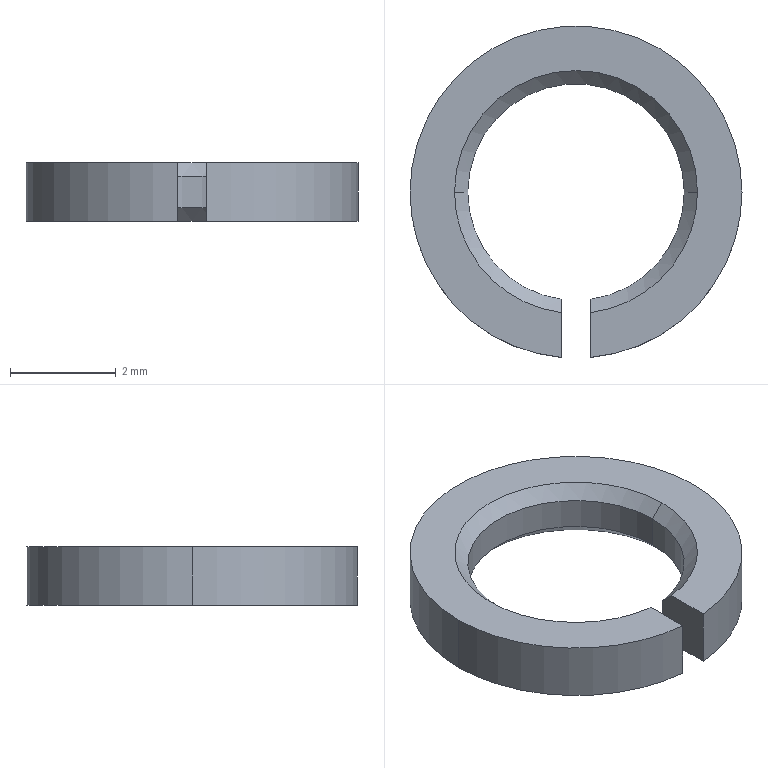Component | SolidWorks | GB_T93-1987StandardTypeSpringWasher4_1.1-6 | 1 solid | 16 faces | box 6.29 x 6.27 x 1.1 mm | volume 18 mm3 | cone 6 | cylinder 6 | plane 4 | commonest cylinder face diameters 4.1 x3 6.287 x3 | material 65Mn
build123d program:
from build123d import *

# Parameters (mm, degrees)
EXTRUDE1_DEPTH = 1.1
CHAMFER1_SIZE  = 0.25


with BuildPart() as part:
    # Sketch1 → Extrude1 (new body)
    with BuildSketch(Plane.XY):
        with BuildLine():
            Line((-0.275, 3.131), (-0.275, 2.031))
            ThreePointArc((-0.275, 2.031), (0, -2.05), (0.275, 2.031))
            Line((0.275, 2.031), (0.275, 3.131))
            ThreePointArc((0.275, 3.131), (0, -3.144), (-0.275, 3.131))
        make_face()
    extrude(amount=EXTRUDE1_DEPTH)

    # Chamfer1
    chamfer1_edges = [part.edges().sort_by_distance(p)[0] for p in [
        (0, -2.05, 1.1),
        (0, -2.05, 0),
    ]]
    chamfer(chamfer1_edges, length=CHAMFER1_SIZE)


solid = part.part

# Placed as in the assembly
solid = solid.moved(Location((58.994, 24.5, 13.9), (180, 0, 0)))
STEP:
#1=COLOUR_RGB('',0.7922,0.8196,0.9333);
#2=FILL_AREA_STYLE_COLOUR('',#1);
#3=FILL_AREA_STYLE('',(#2));
#4=SURFACE_STYLE_FILL_AREA(#3);
#5=SURFACE_SIDE_STYLE('',(#4));
#6=SURFACE_STYLE_USAGE(.BOTH.,#5);
#7=PRESENTATION_STYLE_ASSIGNMENT((#6));
#8=CARTESIAN_POINT('',(2.403,0.9646,0.5374));
#9=VERTEX_POINT('',#8);
#10=CARTESIAN_POINT('',(2.242,0.9646,0.5374));
#11=VERTEX_POINT('',#10);
#12=CARTESIAN_POINT('',(2.323,0.9646,0.5374));
#13=DIRECTION('',(0.,0.,1.));
#14=DIRECTION('',(1.,0.,0.));
#15=AXIS2_PLACEMENT_3D('',#12,#13,#14);
#16=CIRCLE('',#15,0.08071);
#17=EDGE_CURVE('',#9,#11,#16,.T.);
#18=ORIENTED_EDGE('',*,*,#17,.F.);
#19=CARTESIAN_POINT('',(2.413,0.9646,0.5472));
#20=VERTEX_POINT('',#19);
#21=CARTESIAN_POINT('',(2.403,0.9646,0.5374));
#22=DIRECTION('',(0.7071,0.,0.7071));
#23=VECTOR('',#22,39.37);
#24=LINE('',#21,#23);
#25=EDGE_CURVE('',#9,#20,#24,.T.);
#26=ORIENTED_EDGE('',*,*,#25,.T.);
#27=CARTESIAN_POINT('',(2.232,0.9646,0.5472));
#28=VERTEX_POINT('',#27);
#29=CARTESIAN_POINT('',(2.323,0.9646,0.5472));
#30=DIRECTION('',(0.,-0.,-1.));
#31=DIRECTION('',(1.,0.,0.));
#32=AXIS2_PLACEMENT_3D('',#29,#30,#31);
#33=CIRCLE('',#32,0.09055);
#34=EDGE_CURVE('',#28,#20,#33,.T.);
#35=ORIENTED_EDGE('',*,*,#34,.F.);
#36=CARTESIAN_POINT('',(2.242,0.9646,0.5374));
#37=DIRECTION('',(-0.7071,0.,0.7071));
#38=VECTOR('',#37,39.37);
#39=LINE('',#36,#38);
#40=EDGE_CURVE('',#11,#28,#39,.T.);
#41=ORIENTED_EDGE('',*,*,#40,.F.);
#42=EDGE_LOOP('',(#18,#26,#35,#41));
#43=FACE_OUTER_BOUND('',#42,.T.);
#44=CARTESIAN_POINT('',(2.323,0.9646,0.5374));
#45=DIRECTION('',(0.,0.,1.));
#46=DIRECTION('',(-1.,0.,0.));
#47=AXIS2_PLACEMENT_3D('',#44,#45,#46);
#48=CONICAL_SURFACE('',#47,0.08071,0.7854);
#49=ADVANCED_FACE('',(#43),#48,.F.);
#50=CARTESIAN_POINT('',(2.312,0.8846,0.5374));
#51=VERTEX_POINT('',#50);
#52=CARTESIAN_POINT('',(2.323,0.9646,0.5374));
#53=DIRECTION('',(0.,0.,1.));
#54=DIRECTION('',(1.,0.,0.));
#55=AXIS2_PLACEMENT_3D('',#52,#53,#54);
#56=CIRCLE('',#55,0.08071);
#57=EDGE_CURVE('',#11,#51,#56,.T.);
#58=ORIENTED_EDGE('',*,*,#57,.F.);
#59=ORIENTED_EDGE('',*,*,#40,.T.);
#60=CARTESIAN_POINT('',(2.312,0.8747,0.5472));
#61=VERTEX_POINT('',#60);
#62=CARTESIAN_POINT('',(2.323,0.9646,0.5472));
#63=DIRECTION('',(0.,-0.,-1.));
#64=DIRECTION('',(1.,0.,0.));
#65=AXIS2_PLACEMENT_3D('',#62,#63,#64);
#66=CIRCLE('',#65,0.09055);
#67=EDGE_CURVE('',#61,#28,#66,.T.);
#68=ORIENTED_EDGE('',*,*,#67,.F.);
#69=CARTESIAN_POINT('',(2.312,0.8846,0.5374));
#70=CARTESIAN_POINT('',(2.312,0.8813,0.5407));
#71=CARTESIAN_POINT('',(2.312,0.878,0.544));
#72=CARTESIAN_POINT('',(2.312,0.8747,0.5472));
#73=B_SPLINE_CURVE_WITH_KNOTS('',3,(#69,#70,#71,#72),.UNSPECIFIED.,.F.,.F.,(4,4),(0.,0.000355),.UNSPECIFIED.);
#74=EDGE_CURVE('',#51,#61,#73,.T.);
#75=ORIENTED_EDGE('',*,*,#74,.F.);
#76=EDGE_LOOP('',(#58,#59,#68,#75));
#77=FACE_OUTER_BOUND('',#76,.T.);
#78=CARTESIAN_POINT('',(2.323,0.9646,0.5374));
#79=DIRECTION('',(0.,0.,1.));
#80=DIRECTION('',(-1.,0.,0.));
#81=AXIS2_PLACEMENT_3D('',#78,#79,#80);
#82=CONICAL_SURFACE('',#81,0.08071,0.7854);
#83=ADVANCED_FACE('',(#77),#82,.F.);
#84=CARTESIAN_POINT('',(2.242,0.9646,0.5138));
#85=VERTEX_POINT('',#84);
#86=CARTESIAN_POINT('',(2.403,0.9646,0.5138));
#87=VERTEX_POINT('',#86);
#88=CARTESIAN_POINT('',(2.323,0.9646,0.5138));
#89=DIRECTION('',(0.,-0.,-1.));
#90=DIRECTION('',(1.,0.,0.));
#91=AXIS2_PLACEMENT_3D('',#88,#89,#90);
#92=CIRCLE('',#91,0.08071);
#93=EDGE_CURVE('',#85,#87,#92,.T.);
#94=ORIENTED_EDGE('',*,*,#93,.F.);
#95=CARTESIAN_POINT('',(2.232,0.9646,0.5039));
#96=VERTEX_POINT('',#95);
#97=CARTESIAN_POINT('',(2.232,0.9646,0.5039));
#98=DIRECTION('',(-0.7071,-0.,-0.7071));
#99=VECTOR('',#98,39.37);
#100=LINE('',#97,#99);
#101=EDGE_CURVE('',#85,#96,#100,.T.);
#102=ORIENTED_EDGE('',*,*,#101,.T.);
#103=CARTESIAN_POINT('',(2.413,0.9646,0.5039));
#104=VERTEX_POINT('',#103);
#105=CARTESIAN_POINT('',(2.323,0.9646,0.5039));
#106=DIRECTION('',(0.,0.,1.));
#107=DIRECTION('',(1.,0.,0.));
#108=AXIS2_PLACEMENT_3D('',#105,#106,#107);
#109=CIRCLE('',#108,0.09055);
#110=EDGE_CURVE('',#104,#96,#109,.T.);
#111=ORIENTED_EDGE('',*,*,#110,.F.);
#112=CARTESIAN_POINT('',(2.413,0.9646,0.5039));
#113=DIRECTION('',(0.7071,-0.,-0.7071));
#114=VECTOR('',#113,39.37);
#115=LINE('',#112,#114);
#116=EDGE_CURVE('',#87,#104,#115,.T.);
#117=ORIENTED_EDGE('',*,*,#116,.F.);
#118=EDGE_LOOP('',(#94,#102,#111,#117));
#119=FACE_OUTER_BOUND('',#118,.T.);
#120=CARTESIAN_POINT('',(2.323,0.9646,0.5039));
#121=DIRECTION('',(0.,-0.,-1.));
#122=DIRECTION('',(1.,0.,0.));
#123=AXIS2_PLACEMENT_3D('',#120,#121,#122);
#124=CONICAL_SURFACE('',#123,0.09055,0.7854);
#125=ADVANCED_FACE('',(#119),#124,.F.);
#126=CARTESIAN_POINT('',(2.333,0.8846,0.5138));
#127=VERTEX_POINT('',#126);
#128=CARTESIAN_POINT('',(2.323,0.9646,0.5138));
#129=DIRECTION('',(0.,-0.,-1.));
#130=DIRECTION('',(1.,0.,0.));
#131=AXIS2_PLACEMENT_3D('',#128,#129,#130);
#132=CIRCLE('',#131,0.08071);
#133=EDGE_CURVE('',#87,#127,#132,.T.);
#134=ORIENTED_EDGE('',*,*,#133,.F.);
#135=ORIENTED_EDGE('',*,*,#116,.T.);
#136=CARTESIAN_POINT('',(2.333,0.8747,0.5039));
#137=VERTEX_POINT('',#136);
#138=CARTESIAN_POINT('',(2.323,0.9646,0.5039));
#139=DIRECTION('',(0.,0.,1.));
#140=DIRECTION('',(1.,0.,0.));
#141=AXIS2_PLACEMENT_3D('',#138,#139,#140);
#142=CIRCLE('',#141,0.09055);
#143=EDGE_CURVE('',#137,#104,#142,.T.);
#144=ORIENTED_EDGE('',*,*,#143,.F.);
#145=CARTESIAN_POINT('',(2.333,0.8846,0.5138));
#146=CARTESIAN_POINT('',(2.333,0.8813,0.5105));
#147=CARTESIAN_POINT('',(2.333,0.878,0.5072));
#148=CARTESIAN_POINT('',(2.333,0.8747,0.5039));
#149=B_SPLINE_CURVE_WITH_KNOTS('',3,(#145,#146,#147,#148),.UNSPECIFIED.,.F.,.F.,(4,4),(0.,0.000355),.UNSPECIFIED.);
#150=EDGE_CURVE('',#127,#137,#149,.T.);
#151=ORIENTED_EDGE('',*,*,#150,.F.);
#152=EDGE_LOOP('',(#134,#135,#144,#151));
#153=FACE_OUTER_BOUND('',#152,.T.);
#154=CARTESIAN_POINT('',(2.323,0.9646,0.5039));
#155=DIRECTION('',(0.,-0.,-1.));
#156=DIRECTION('',(1.,0.,0.));
#157=AXIS2_PLACEMENT_3D('',#154,#155,#156);
#158=CONICAL_SURFACE('',#157,0.09055,0.7854);
#159=ADVANCED_FACE('',(#153),#158,.F.);
#160=ORIENTED_EDGE('',*,*,#93,.T.);
#161=CARTESIAN_POINT('',(2.403,0.9646,0.5039));
#162=DIRECTION('',(0.,0.,1.));
#163=VECTOR('',#162,39.37);
#164=LINE('',#161,#163);
#165=EDGE_CURVE('',#87,#9,#164,.T.);
#166=ORIENTED_EDGE('',*,*,#165,.T.);
#167=ORIENTED_EDGE('',*,*,#17,.T.);
#168=CARTESIAN_POINT('',(2.242,0.9646,0.5039));
#169=DIRECTION('',(0.,0.,1.));
#170=VECTOR('',#169,39.37);
#171=LINE('',#168,#170);
#172=EDGE_CURVE('',#85,#11,#171,.T.);
#173=ORIENTED_EDGE('',*,*,#172,.F.);
#174=EDGE_LOOP('',(#160,#166,#167,#173));
#175=FACE_OUTER_BOUND('',#174,.T.);
#176=CARTESIAN_POINT('',(2.323,0.9646,0.5039));
#177=DIRECTION('',(0.,0.,1.));
#178=DIRECTION('',(-1.,0.,0.));
#179=AXIS2_PLACEMENT_3D('',#176,#177,#178);
#180=CYLINDRICAL_SURFACE('',#179,0.08071);
#181=ADVANCED_FACE('',(#175),#180,.F.);
#182=CARTESIAN_POINT('',(2.312,0.8846,0.5138));
#183=VERTEX_POINT('',#182);
#184=CARTESIAN_POINT('',(2.323,0.9646,0.5138));
#185=DIRECTION('',(0.,-0.,-1.));
#186=DIRECTION('',(1.,0.,0.));
#187=AXIS2_PLACEMENT_3D('',#184,#185,#186);
#188=CIRCLE('',#187,0.08071);
#189=EDGE_CURVE('',#183,#85,#188,.T.);
#190=ORIENTED_EDGE('',*,*,#189,.T.);
#191=ORIENTED_EDGE('',*,*,#172,.T.);
#192=ORIENTED_EDGE('',*,*,#57,.T.);
#193=CARTESIAN_POINT('',(2.312,0.8846,0.5039));
#194=DIRECTION('',(0.,0.,1.));
#195=VECTOR('',#194,39.37);
#196=LINE('',#193,#195);
#197=EDGE_CURVE('',#183,#51,#196,.T.);
#198=ORIENTED_EDGE('',*,*,#197,.F.);
#199=EDGE_LOOP('',(#190,#191,#192,#198));
#200=FACE_OUTER_BOUND('',#199,.T.);
#201=CARTESIAN_POINT('',(2.323,0.9646,0.5039));
#202=DIRECTION('',(0.,0.,1.));
#203=DIRECTION('',(-1.,0.,0.));
#204=AXIS2_PLACEMENT_3D('',#201,#202,#203);
#205=CYLINDRICAL_SURFACE('',#204,0.08071);
#206=ADVANCED_FACE('',(#200),#205,.F.);
#207=CARTESIAN_POINT('',(2.446,0.9646,0.5039));
#208=VERTEX_POINT('',#207);
#209=CARTESIAN_POINT('',(2.333,0.8413,0.5039));
#210=VERTEX_POINT('',#209);
#211=CARTESIAN_POINT('',(2.323,0.9646,0.5039));
#212=DIRECTION('',(0.,-0.,-1.));
#213=DIRECTION('',(1.,0.,0.));
#214=AXIS2_PLACEMENT_3D('',#211,#212,#213);
#215=CIRCLE('',#214,0.1238);
#216=EDGE_CURVE('',#208,#210,#215,.T.);
#217=ORIENTED_EDGE('',*,*,#216,.F.);
#218=CARTESIAN_POINT('',(2.446,0.9646,0.5472));
#219=VERTEX_POINT('',#218);
#220=CARTESIAN_POINT('',(2.446,0.9646,0.5039));
#221=DIRECTION('',(0.,0.,1.));
#222=VECTOR('',#221,39.37);
#223=LINE('',#220,#222);
#224=EDGE_CURVE('',#208,#219,#223,.T.);
#225=ORIENTED_EDGE('',*,*,#224,.T.);
#226=CARTESIAN_POINT('',(2.333,0.8413,0.5472));
#227=VERTEX_POINT('',#226);
#228=CARTESIAN_POINT('',(2.323,0.9646,0.5472));
#229=DIRECTION('',(0.,-0.,-1.));
#230=DIRECTION('',(1.,0.,0.));
#231=AXIS2_PLACEMENT_3D('',#228,#229,#230);
#232=CIRCLE('',#231,0.1238);
#233=EDGE_CURVE('',#219,#227,#232,.T.);
#234=ORIENTED_EDGE('',*,*,#233,.T.);
#235=CARTESIAN_POINT('',(2.333,0.8413,0.5039));
#236=DIRECTION('',(0.,0.,1.));
#237=VECTOR('',#236,39.37);
#238=LINE('',#235,#237);
#239=EDGE_CURVE('',#210,#227,#238,.T.);
#240=ORIENTED_EDGE('',*,*,#239,.F.);
#241=EDGE_LOOP('',(#217,#225,#234,#240));
#242=FACE_OUTER_BOUND('',#241,.T.);
#243=CARTESIAN_POINT('',(2.323,0.9646,0.5039));
#244=DIRECTION('',(0.,0.,1.));
#245=DIRECTION('',(-1.,0.,0.));
#246=AXIS2_PLACEMENT_3D('',#243,#244,#245);
#247=CYLINDRICAL_SURFACE('',#246,0.1238);
#248=ADVANCED_FACE('',(#242),#247,.T.);
#249=ORIENTED_EDGE('',*,*,#224,.F.);
#250=CARTESIAN_POINT('',(2.199,0.9646,0.5039));
#251=VERTEX_POINT('',#250);
#252=CARTESIAN_POINT('',(2.323,0.9646,0.5039));
#253=DIRECTION('',(0.,-0.,-1.));
#254=DIRECTION('',(1.,0.,0.));
#255=AXIS2_PLACEMENT_3D('',#252,#253,#254);
#256=CIRCLE('',#255,0.1238);
#257=EDGE_CURVE('',#251,#208,#256,.T.);
#258=ORIENTED_EDGE('',*,*,#257,.F.);
#259=CARTESIAN_POINT('',(2.199,0.9646,0.5472));
#260=VERTEX_POINT('',#259);
#261=CARTESIAN_POINT('',(2.199,0.9646,0.5039));
#262=DIRECTION('',(0.,0.,1.));
#263=VECTOR('',#262,39.37);
#264=LINE('',#261,#263);
#265=EDGE_CURVE('',#251,#260,#264,.T.);
#266=ORIENTED_EDGE('',*,*,#265,.T.);
#267=CARTESIAN_POINT('',(2.323,0.9646,0.5472));
#268=DIRECTION('',(0.,-0.,-1.));
#269=DIRECTION('',(1.,0.,0.));
#270=AXIS2_PLACEMENT_3D('',#267,#268,#269);
#271=CIRCLE('',#270,0.1238);
#272=EDGE_CURVE('',#260,#219,#271,.T.);
#273=ORIENTED_EDGE('',*,*,#272,.T.);
#274=EDGE_LOOP('',(#249,#258,#266,#273));
#275=FACE_OUTER_BOUND('',#274,.T.);
#276=CARTESIAN_POINT('',(2.323,0.9646,0.5039));
#277=DIRECTION('',(0.,0.,1.));
#278=DIRECTION('',(-1.,0.,0.));
#279=AXIS2_PLACEMENT_3D('',#276,#277,#278);
#280=CYLINDRICAL_SURFACE('',#279,0.1238);
#281=ADVANCED_FACE('',(#275),#280,.T.);
#282=ORIENTED_EDGE('',*,*,#265,.F.);
#283=CARTESIAN_POINT('',(2.312,0.8413,0.5039));
#284=VERTEX_POINT('',#283);
#285=CARTESIAN_POINT('',(2.323,0.9646,0.5039));
#286=DIRECTION('',(0.,-0.,-1.));
#287=DIRECTION('',(1.,0.,0.));
#288=AXIS2_PLACEMENT_3D('',#285,#286,#287);
#289=CIRCLE('',#288,0.1238);
#290=EDGE_CURVE('',#284,#251,#289,.T.);
#291=ORIENTED_EDGE('',*,*,#290,.F.);
#292=CARTESIAN_POINT('',(2.312,0.8413,0.5472));
#293=VERTEX_POINT('',#292);
#294=CARTESIAN_POINT('',(2.312,0.8413,0.5039));
#295=DIRECTION('',(0.,0.,1.));
#296=VECTOR('',#295,39.37);
#297=LINE('',#294,#296);
#298=EDGE_CURVE('',#284,#293,#297,.T.);
#299=ORIENTED_EDGE('',*,*,#298,.T.);
#300=CARTESIAN_POINT('',(2.323,0.9646,0.5472));
#301=DIRECTION('',(0.,-0.,-1.));
#302=DIRECTION('',(1.,0.,0.));
#303=AXIS2_PLACEMENT_3D('',#300,#301,#302);
#304=CIRCLE('',#303,0.1238);
#305=EDGE_CURVE('',#293,#260,#304,.T.);
#306=ORIENTED_EDGE('',*,*,#305,.T.);
#307=EDGE_LOOP('',(#282,#291,#299,#306));
#308=FACE_OUTER_BOUND('',#307,.T.);
#309=CARTESIAN_POINT('',(2.323,0.9646,0.5039));
#310=DIRECTION('',(0.,0.,1.));
#311=DIRECTION('',(-1.,0.,0.));
#312=AXIS2_PLACEMENT_3D('',#309,#310,#311);
#313=CYLINDRICAL_SURFACE('',#312,0.1238);
#314=ADVANCED_FACE('',(#308),#313,.T.);
#315=CARTESIAN_POINT('',(2.333,0.8846,0.5374));
#316=VERTEX_POINT('',#315);
#317=CARTESIAN_POINT('',(2.333,0.8846,0.5039));
#318=DIRECTION('',(0.,0.,1.));
#319=VECTOR('',#318,39.37);
#320=LINE('',#317,#319);
#321=EDGE_CURVE('',#127,#316,#320,.T.);
#322=ORIENTED_EDGE('',*,*,#321,.F.);
#323=ORIENTED_EDGE('',*,*,#150,.T.);
#324=CARTESIAN_POINT('',(2.333,0.8413,0.5039));
#325=DIRECTION('',(0.,1.,-0.));
#326=VECTOR('',#325,39.37);
#327=LINE('',#324,#326);
#328=EDGE_CURVE('',#210,#137,#327,.T.);
#329=ORIENTED_EDGE('',*,*,#328,.F.);
#330=ORIENTED_EDGE('',*,*,#239,.T.);
#331=CARTESIAN_POINT('',(2.333,0.8747,0.5472));
#332=VERTEX_POINT('',#331);
#333=CARTESIAN_POINT('',(2.333,0.8413,0.5472));
#334=DIRECTION('',(0.,1.,-0.));
#335=VECTOR('',#334,39.37);
#336=LINE('',#333,#335);
#337=EDGE_CURVE('',#227,#332,#336,.T.);
#338=ORIENTED_EDGE('',*,*,#337,.T.);
#339=CARTESIAN_POINT('',(2.333,0.8747,0.5472));
#340=CARTESIAN_POINT('',(2.333,0.878,0.544));
#341=CARTESIAN_POINT('',(2.333,0.8813,0.5407));
#342=CARTESIAN_POINT('',(2.333,0.8846,0.5374));
#343=B_SPLINE_CURVE_WITH_KNOTS('',3,(#339,#340,#341,#342),.UNSPECIFIED.,.F.,.F.,(4,4),(0.,0.000355),.UNSPECIFIED.);
#344=EDGE_CURVE('',#332,#316,#343,.T.);
#345=ORIENTED_EDGE('',*,*,#344,.T.);
#346=EDGE_LOOP('',(#322,#323,#329,#330,#338,#345));
#347=FACE_OUTER_BOUND('',#346,.T.);
#348=CARTESIAN_POINT('',(2.333,0.8413,0.5039));
#349=DIRECTION('',(1.,0.,0.));
#350=DIRECTION('',(0.,0.,1.));
#351=AXIS2_PLACEMENT_3D('',#348,#349,#350);
#352=PLANE('',#351);
#353=ADVANCED_FACE('',(#347),#352,.F.);
#354=ORIENTED_EDGE('',*,*,#165,.F.);
#355=ORIENTED_EDGE('',*,*,#133,.T.);
#356=ORIENTED_EDGE('',*,*,#321,.T.);
#357=CARTESIAN_POINT('',(2.323,0.9646,0.5374));
#358=DIRECTION('',(0.,0.,1.));
#359=DIRECTION('',(1.,0.,0.));
#360=AXIS2_PLACEMENT_3D('',#357,#358,#359);
#361=CIRCLE('',#360,0.08071);
#362=EDGE_CURVE('',#316,#9,#361,.T.);
#363=ORIENTED_EDGE('',*,*,#362,.T.);
#364=EDGE_LOOP('',(#354,#355,#356,#363));
#365=FACE_OUTER_BOUND('',#364,.T.);
#366=CARTESIAN_POINT('',(2.323,0.9646,0.5039));
#367=DIRECTION('',(0.,0.,1.));
#368=DIRECTION('',(-1.,0.,0.));
#369=AXIS2_PLACEMENT_3D('',#366,#367,#368);
#370=CYLINDRICAL_SURFACE('',#369,0.08071);
#371=ADVANCED_FACE('',(#365),#370,.F.);
#372=CARTESIAN_POINT('',(2.312,0.8747,0.5039));
#373=VERTEX_POINT('',#372);
#374=CARTESIAN_POINT('',(2.312,0.8413,0.5039));
#375=DIRECTION('',(0.,-1.,0.));
#376=VECTOR('',#375,39.37);
#377=LINE('',#374,#376);
#378=EDGE_CURVE('',#373,#284,#377,.T.);
#379=ORIENTED_EDGE('',*,*,#378,.F.);
#380=CARTESIAN_POINT('',(2.312,0.8747,0.5039));
#381=CARTESIAN_POINT('',(2.312,0.878,0.5072));
#382=CARTESIAN_POINT('',(2.312,0.8813,0.5105));
#383=CARTESIAN_POINT('',(2.312,0.8846,0.5138));
#384=B_SPLINE_CURVE_WITH_KNOTS('',3,(#380,#381,#382,#383),.UNSPECIFIED.,.F.,.F.,(4,4),(0.,0.000355),.UNSPECIFIED.);
#385=EDGE_CURVE('',#373,#183,#384,.T.);
#386=ORIENTED_EDGE('',*,*,#385,.T.);
#387=ORIENTED_EDGE('',*,*,#197,.T.);
#388=ORIENTED_EDGE('',*,*,#74,.T.);
#389=CARTESIAN_POINT('',(2.312,0.8413,0.5472));
#390=DIRECTION('',(0.,-1.,0.));
#391=VECTOR('',#390,39.37);
#392=LINE('',#389,#391);
#393=EDGE_CURVE('',#61,#293,#392,.T.);
#394=ORIENTED_EDGE('',*,*,#393,.T.);
#395=ORIENTED_EDGE('',*,*,#298,.F.);
#396=EDGE_LOOP('',(#379,#386,#387,#388,#394,#395));
#397=FACE_OUTER_BOUND('',#396,.T.);
#398=CARTESIAN_POINT('',(2.312,0.8413,0.5039));
#399=DIRECTION('',(-1.,0.,0.));
#400=DIRECTION('',(0.,-0.,-1.));
#401=AXIS2_PLACEMENT_3D('',#398,#399,#400);
#402=PLANE('',#401);
#403=ADVANCED_FACE('',(#397),#402,.F.);
#404=ORIENTED_EDGE('',*,*,#328,.T.);
#405=ORIENTED_EDGE('',*,*,#143,.T.);
#406=ORIENTED_EDGE('',*,*,#110,.T.);
#407=CARTESIAN_POINT('',(2.323,0.9646,0.5039));
#408=DIRECTION('',(0.,0.,1.));
#409=DIRECTION('',(1.,0.,0.));
#410=AXIS2_PLACEMENT_3D('',#407,#408,#409);
#411=CIRCLE('',#410,0.09055);
#412=EDGE_CURVE('',#96,#373,#411,.T.);
#413=ORIENTED_EDGE('',*,*,#412,.T.);
#414=ORIENTED_EDGE('',*,*,#378,.T.);
#415=ORIENTED_EDGE('',*,*,#290,.T.);
#416=ORIENTED_EDGE('',*,*,#257,.T.);
#417=ORIENTED_EDGE('',*,*,#216,.T.);
#418=EDGE_LOOP('',(#404,#405,#406,#413,#414,#415,#416,#417));
#419=FACE_OUTER_BOUND('',#418,.T.);
#420=CARTESIAN_POINT('',(2.323,0.9646,0.5039));
#421=DIRECTION('',(0.,-0.,-1.));
#422=DIRECTION('',(1.,0.,0.));
#423=AXIS2_PLACEMENT_3D('',#420,#421,#422);
#424=PLANE('',#423);
#425=ADVANCED_FACE('',(#419),#424,.T.);
#426=ORIENTED_EDGE('',*,*,#393,.F.);
#427=ORIENTED_EDGE('',*,*,#67,.T.);
#428=ORIENTED_EDGE('',*,*,#34,.T.);
#429=CARTESIAN_POINT('',(2.323,0.9646,0.5472));
#430=DIRECTION('',(0.,-0.,-1.));
#431=DIRECTION('',(1.,0.,0.));
#432=AXIS2_PLACEMENT_3D('',#429,#430,#431);
#433=CIRCLE('',#432,0.09055);
#434=EDGE_CURVE('',#20,#332,#433,.T.);
#435=ORIENTED_EDGE('',*,*,#434,.T.);
#436=ORIENTED_EDGE('',*,*,#337,.F.);
#437=ORIENTED_EDGE('',*,*,#233,.F.);
#438=ORIENTED_EDGE('',*,*,#272,.F.);
#439=ORIENTED_EDGE('',*,*,#305,.F.);
#440=EDGE_LOOP('',(#426,#427,#428,#435,#436,#437,#438,#439));
#441=FACE_OUTER_BOUND('',#440,.T.);
#442=CARTESIAN_POINT('',(2.323,0.9646,0.5472));
#443=DIRECTION('',(0.,-0.,-1.));
#444=DIRECTION('',(1.,0.,0.));
#445=AXIS2_PLACEMENT_3D('',#442,#443,#444);
#446=PLANE('',#445);
#447=ADVANCED_FACE('',(#441),#446,.F.);
#448=ORIENTED_EDGE('',*,*,#101,.F.);
#449=ORIENTED_EDGE('',*,*,#189,.F.);
#450=ORIENTED_EDGE('',*,*,#385,.F.);
#451=ORIENTED_EDGE('',*,*,#412,.F.);
#452=EDGE_LOOP('',(#448,#449,#450,#451));
#453=FACE_OUTER_BOUND('',#452,.T.);
#454=CARTESIAN_POINT('',(2.323,0.9646,0.5039));
#455=DIRECTION('',(0.,-0.,-1.));
#456=DIRECTION('',(1.,0.,0.));
#457=AXIS2_PLACEMENT_3D('',#454,#455,#456);
#458=CONICAL_SURFACE('',#457,0.09055,0.7854);
#459=ADVANCED_FACE('',(#453),#458,.F.);
#460=ORIENTED_EDGE('',*,*,#25,.F.);
#461=ORIENTED_EDGE('',*,*,#362,.F.);
#462=ORIENTED_EDGE('',*,*,#344,.F.);
#463=ORIENTED_EDGE('',*,*,#434,.F.);
#464=EDGE_LOOP('',(#460,#461,#462,#463));
#465=FACE_OUTER_BOUND('',#464,.T.);
#466=CARTESIAN_POINT('',(2.323,0.9646,0.5374));
#467=DIRECTION('',(0.,0.,1.));
#468=DIRECTION('',(-1.,0.,0.));
#469=AXIS2_PLACEMENT_3D('',#466,#467,#468);
#470=CONICAL_SURFACE('',#469,0.08071,0.7854);
#471=ADVANCED_FACE('',(#465),#470,.F.);
#472=CLOSED_SHELL('',(#49,#83,#125,#159,#181,#206,#248,#281,#314,#353,#371,#403,#425,#447,#459,#471));
#473=MANIFOLD_SOLID_BREP('',#472);
#474=STYLED_ITEM('',(#7),#473);
#475=PRESENTATION_LAYER_ASSIGNMENT('','',(#474));
#476=(LENGTH_UNIT()NAMED_UNIT(*)SI_UNIT($,.METRE.));
#477=LENGTH_MEASURE_WITH_UNIT(LENGTH_MEASURE(0.0254),#476);
#478=DIMENSIONAL_EXPONENTS(1.,0.,0.,0.,0.,0.,0.);
#479=(CONVERSION_BASED_UNIT('',#477)LENGTH_UNIT()NAMED_UNIT(#478));
#480=UNCERTAINTY_MEASURE_WITH_UNIT(LENGTH_MEASURE(0.00001),#479,'','');
#481=(NAMED_UNIT(*)PLANE_ANGLE_UNIT()SI_UNIT($,.RADIAN.));
#482=(NAMED_UNIT(*)SI_UNIT($,.STERADIAN.)SOLID_ANGLE_UNIT());
#483=(GEOMETRIC_REPRESENTATION_CONTEXT(3)GLOBAL_UNCERTAINTY_ASSIGNED_CONTEXT((#480))GLOBAL_UNIT_ASSIGNED_CONTEXT((#479,#481,#482))REPRESENTATION_CONTEXT('',''));
#484=MECHANICAL_DESIGN_GEOMETRIC_PRESENTATION_REPRESENTATION('',(#474),#483);
#485=CARTESIAN_POINT('',(0.,0.,0.));
#486=DIRECTION('',(0.,0.,1.));
#487=DIRECTION('',(1.,0.,0.));
#488=AXIS2_PLACEMENT_3D('',#485,#486,#487);
#489=(LENGTH_UNIT()NAMED_UNIT(*)SI_UNIT($,.METRE.));
#490=LENGTH_MEASURE_WITH_UNIT(LENGTH_MEASURE(0.0254),#489);
#491=DIMENSIONAL_EXPONENTS(1.,0.,0.,0.,0.,0.,0.);
#492=(CONVERSION_BASED_UNIT('',#490)LENGTH_UNIT()NAMED_UNIT(#491));
#493=UNCERTAINTY_MEASURE_WITH_UNIT(LENGTH_MEASURE(0.00001),#492,'','');
#494=(NAMED_UNIT(*)PLANE_ANGLE_UNIT()SI_UNIT($,.RADIAN.));
#495=(NAMED_UNIT(*)SI_UNIT($,.STERADIAN.)SOLID_ANGLE_UNIT());
#496=(GEOMETRIC_REPRESENTATION_CONTEXT(3)GLOBAL_UNCERTAINTY_ASSIGNED_CONTEXT((#493))GLOBAL_UNIT_ASSIGNED_CONTEXT((#492,#494,#495))REPRESENTATION_CONTEXT('',''));
#497=ADVANCED_BREP_SHAPE_REPRESENTATION('',(#473,#488),#496);